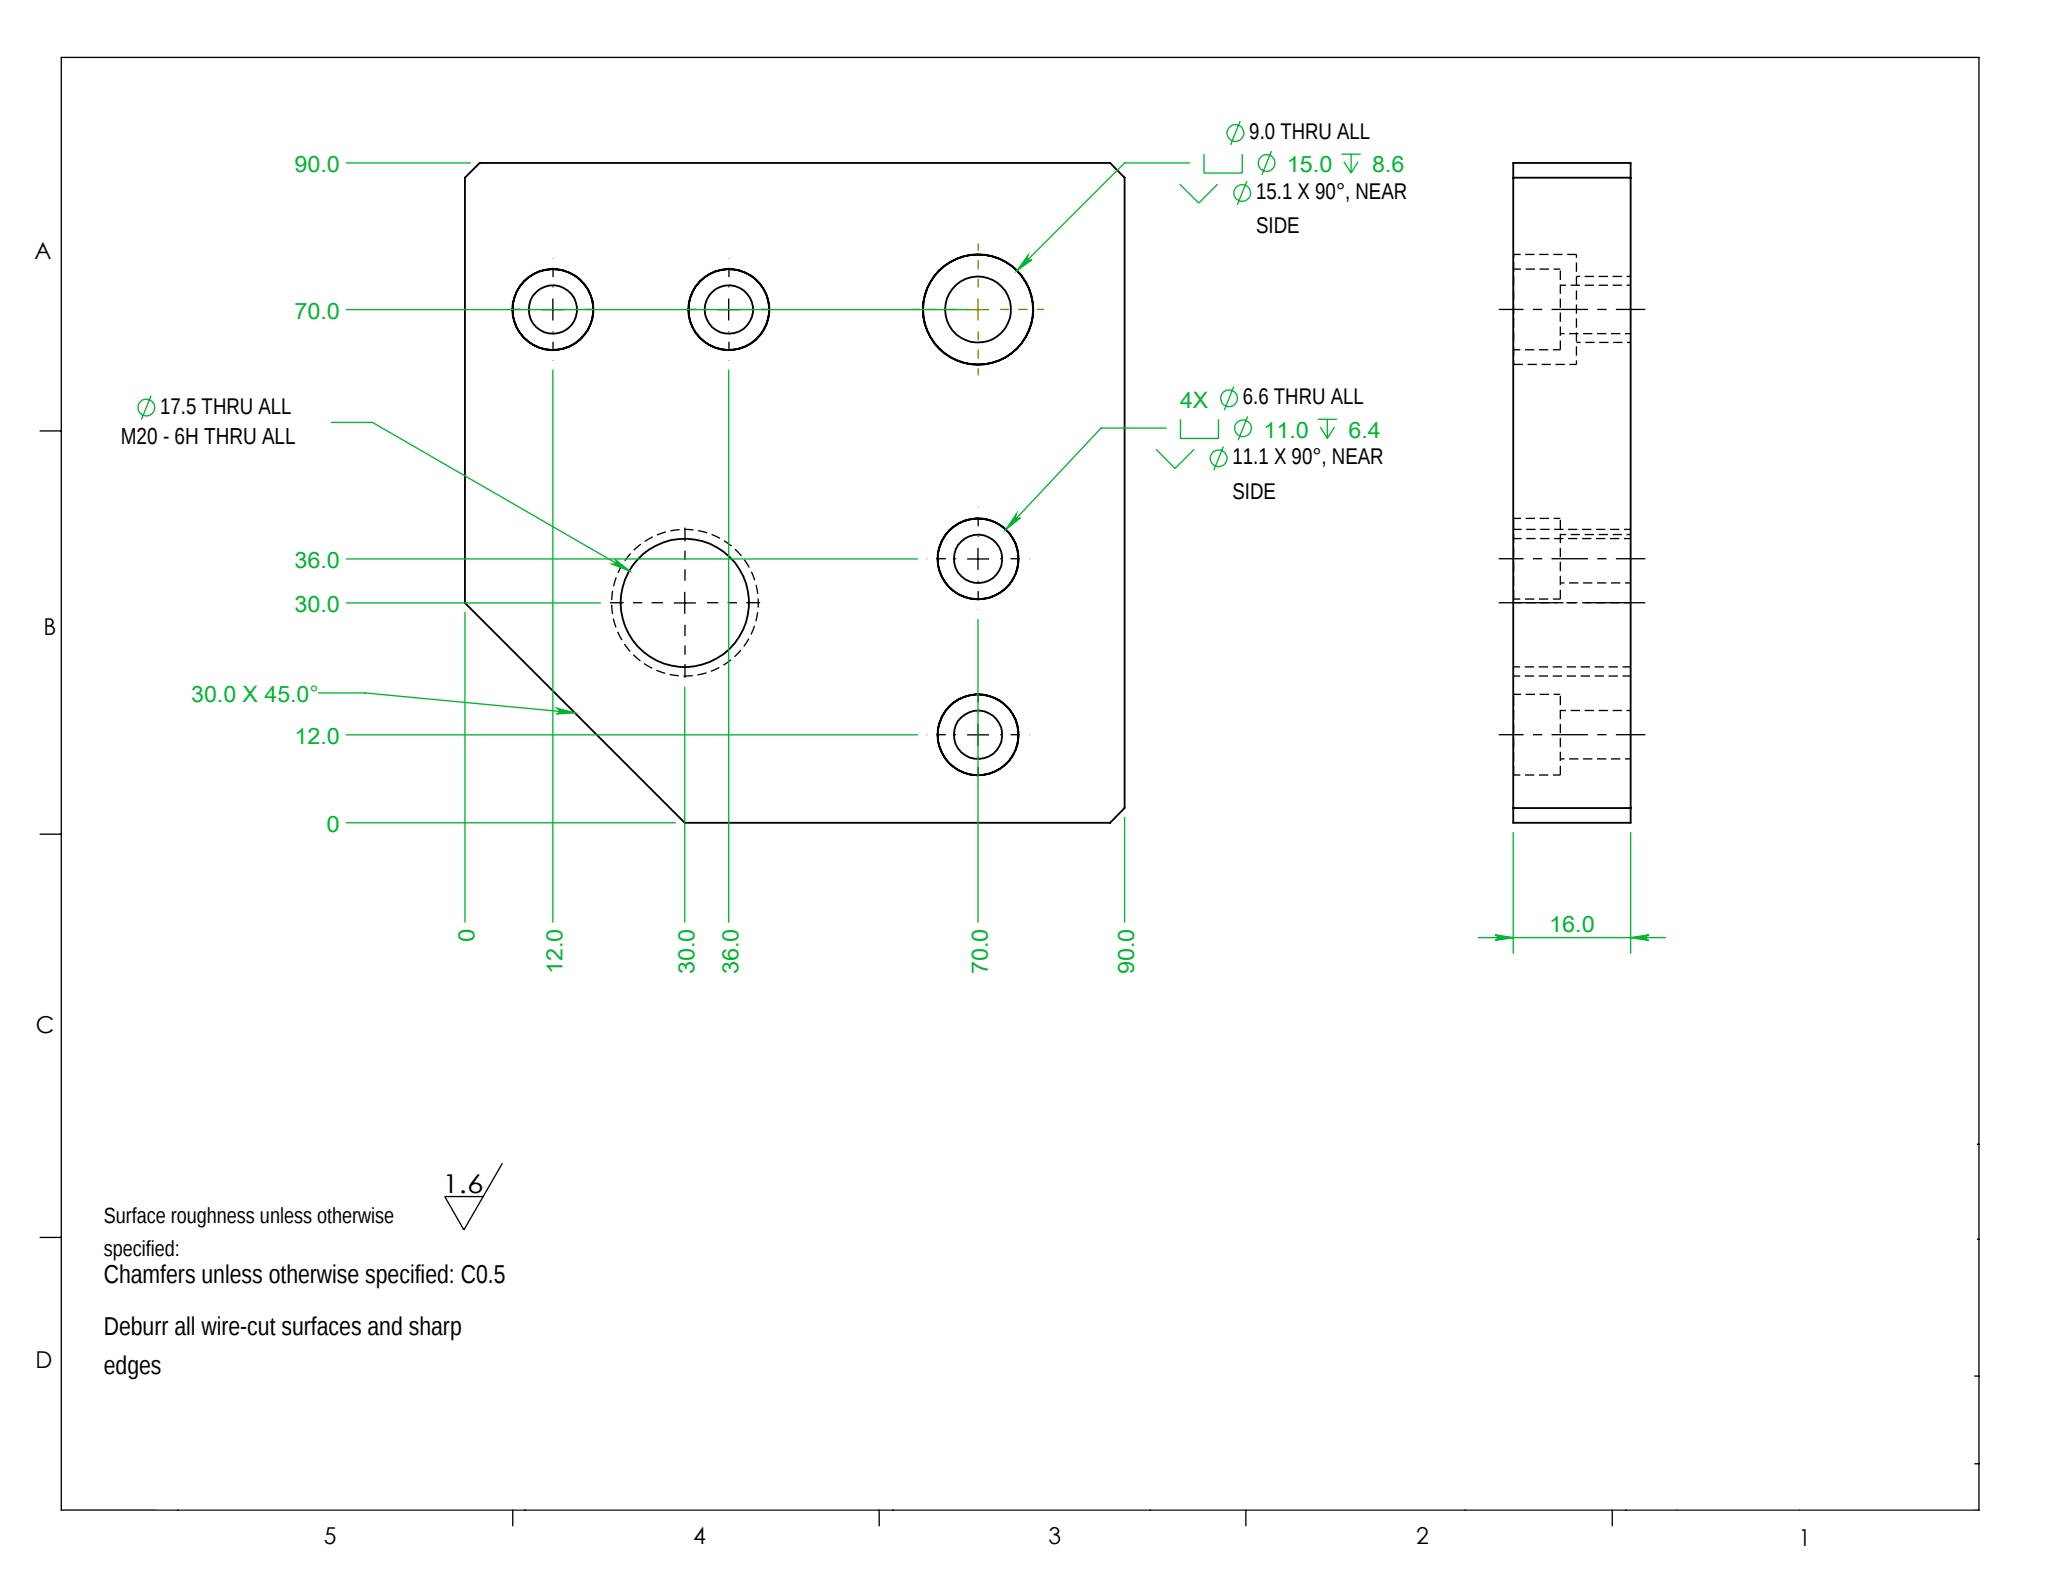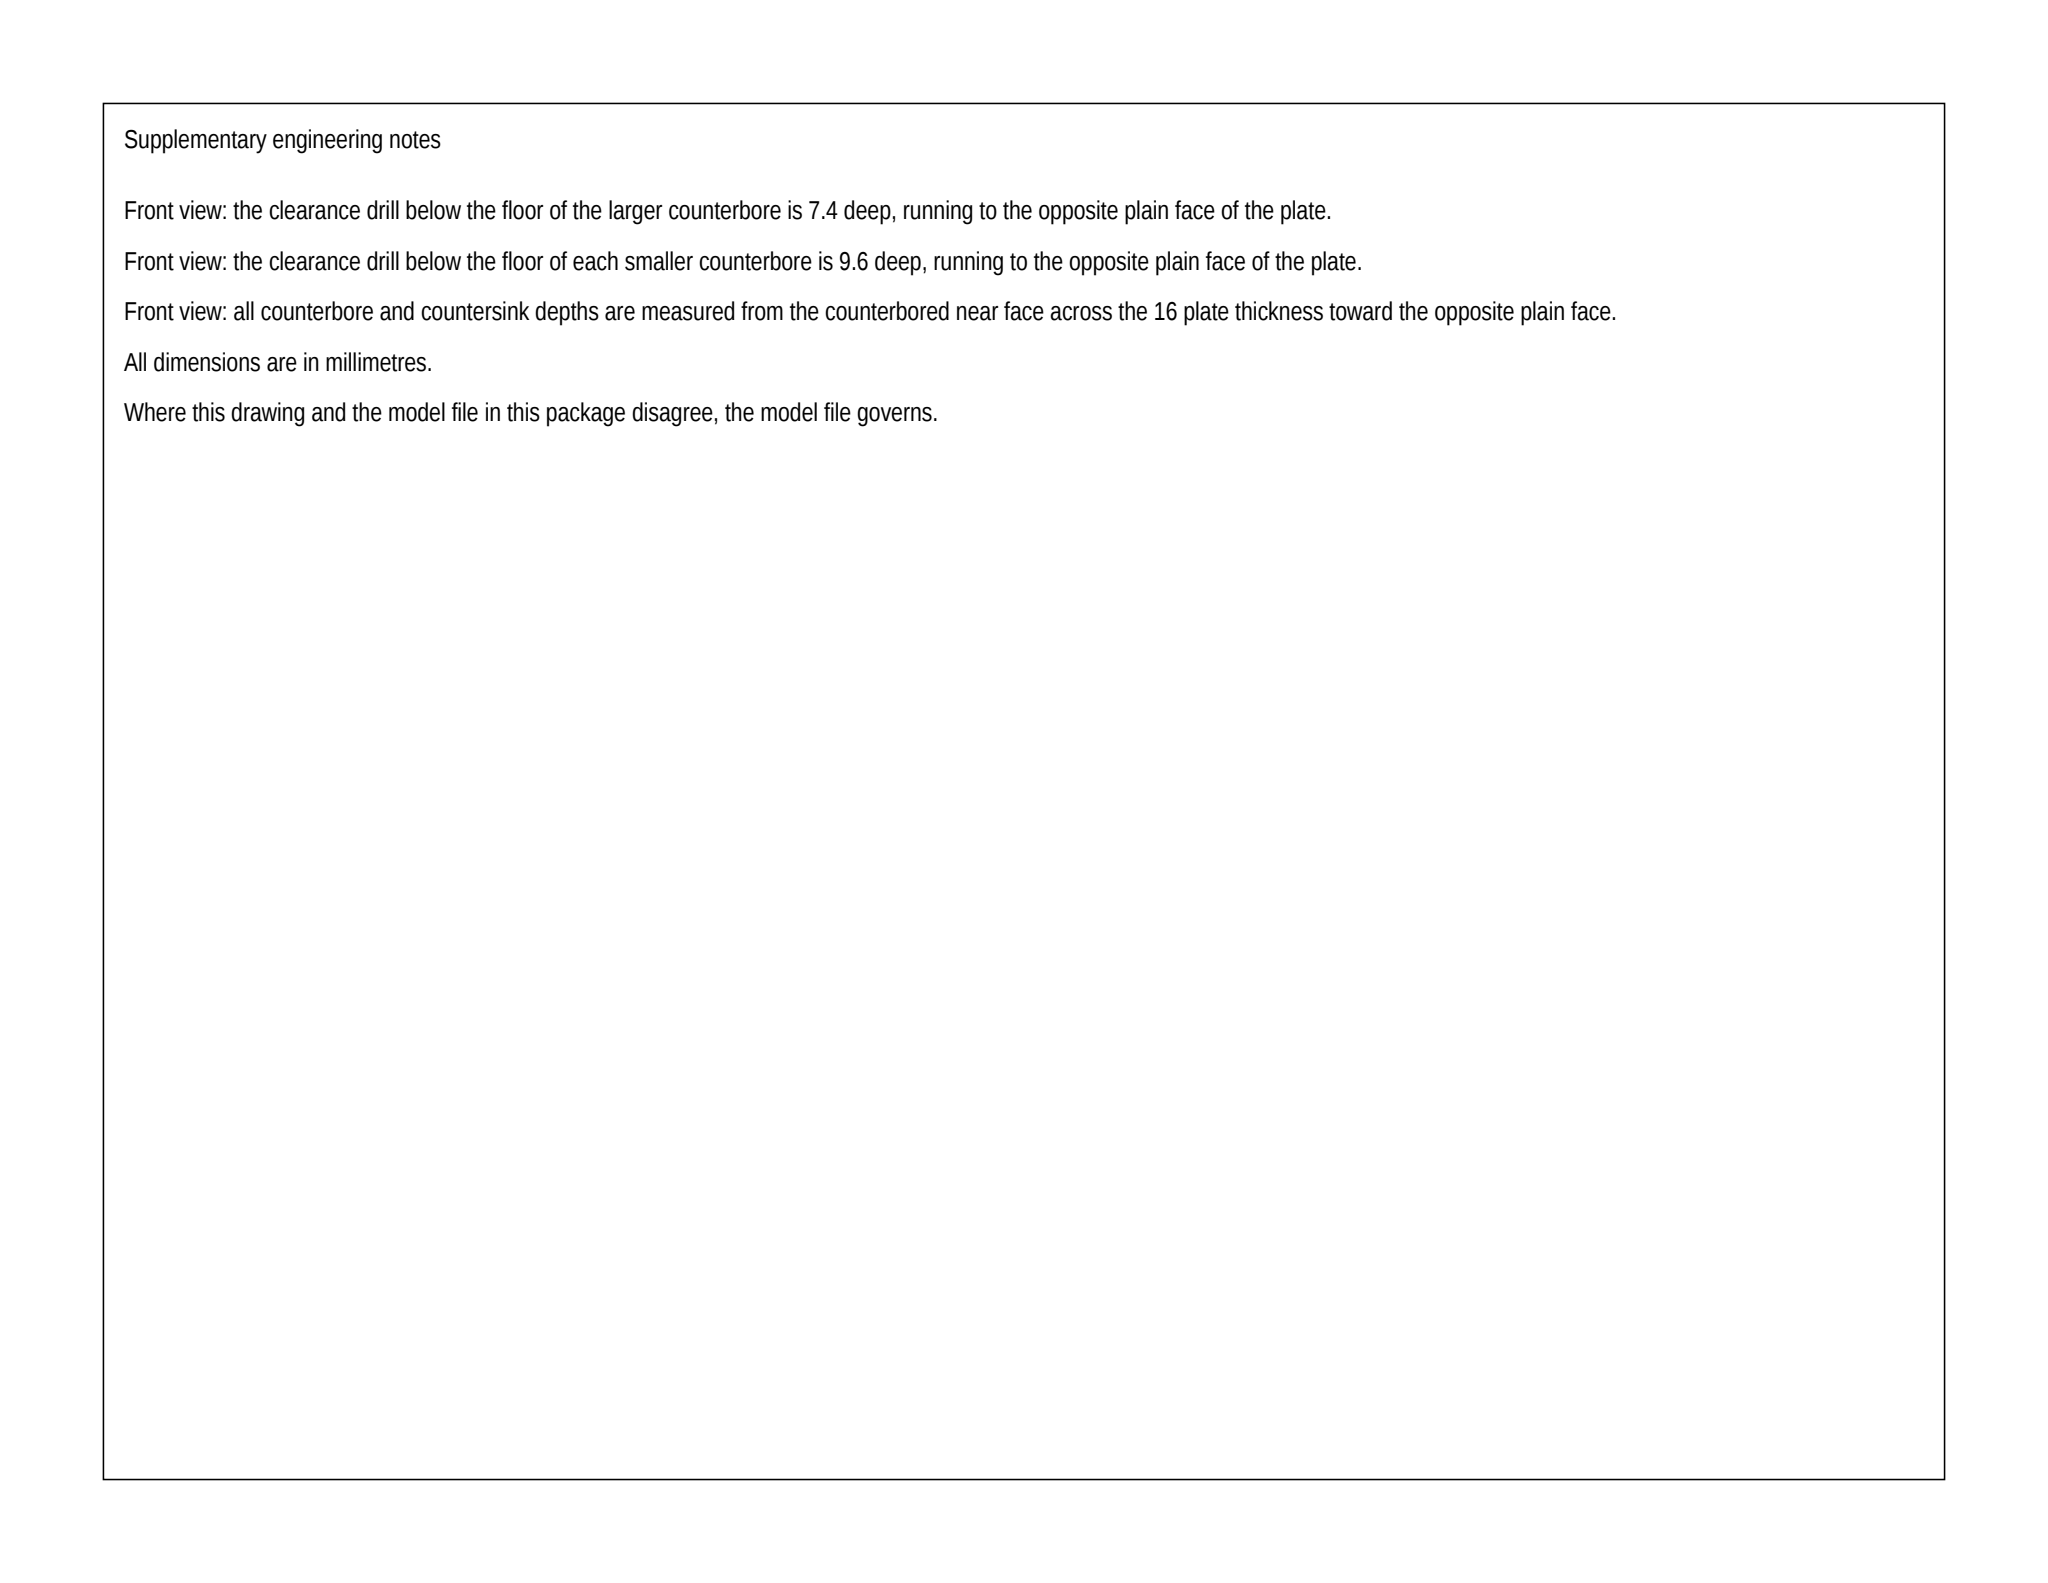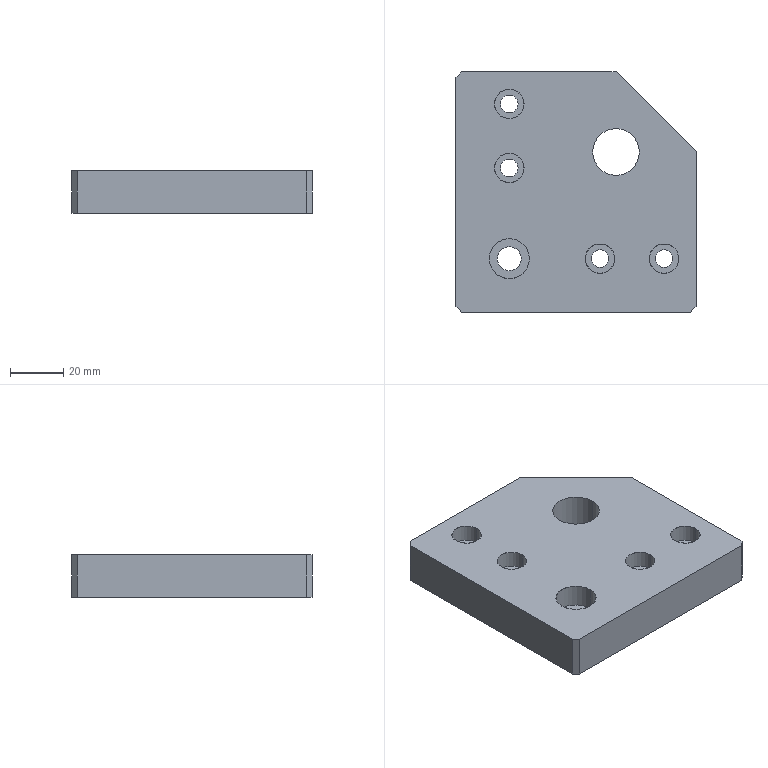Part | SolidWorks | mm | 1 solid | 47 faces | box 90 x 90 x 16 mm | volume 112718 mm3 | cylinder 22 | plane 15 | cone 10 | commonest cylinder face diameters 11 x8 6.6 x8 15 x2 9 x2 17.5 x2
build123d program:
from build123d import *

# Parameters (mm, degrees)
SKETCH1_W                                      = 90
SKETCH1_H                                      = 90
BOSS_EXTRUDE1_DEPTH                            = 16
M6_HEX_SOCKET_HEAD_CAP_SCREW_CBORE1_AT_2_COUNT = 2
M6_HEX_SOCKET_HEAD_CAP_SCREW_CBORE1_AT_2_PITCH = 48.083
M6_HEX_SOCKET_HEAD_CAP_SCREW_CBORE1_AT_3_COUNT = 2
M6_HEX_SOCKET_HEAD_CAP_SCREW_CBORE1_AT_3_PITCH = 67.231
M6_HEX_SOCKET_HEAD_CAP_SCREW_CBORE1_AT_4_COUNT = 2
M6_HEX_SOCKET_HEAD_CAP_SCREW_CBORE1_AT_4_PITCH = 24
CHAMFER1_SIZE                                  = 2
M20_TAPPED_HOLE1_D                             = 17.5
CHAMFER3_SIZE                                  = 30


with BuildPart() as part:
    # Sketch1 → Boss-Extrude1 (new body)
    with BuildSketch(Plane.XY):
        with Locations((45, 45)):
            Rectangle(SKETCH1_W, SKETCH1_H)
    extrude(amount=BOSS_EXTRUDE1_DEPTH)

    # Sketch3 → M6 Hex Socket Head Cap Screw CBORE1 (revolve, cut)
    with BuildSketch(Plane(origin=(20, 54, 16), x_dir=(0, -1, 0), z_dir=(1, 0, 0))):
        Polygon((0, 0), (0, 16), (3.3, 16), (3.3, 6.4), (5.5, 6.4), (5.5, 0.025), (5.525, 0), align=None)
    m6_hex_socket_head_cap_screw_cbore1 = revolve(axis=Axis((20, 54, 22.35), (0, 0, -1)), mode=Mode.SUBTRACT)

    # M6 Hex Socket Head Cap Screw CBORE1 at 2: M6 Hex Socket Head Cap Screw CBORE1 ×2
    with Locations(*[Vector(0.7071, -0.7071, 0) * (i * M6_HEX_SOCKET_HEAD_CAP_SCREW_CBORE1_AT_2_PITCH) for i in range(1, M6_HEX_SOCKET_HEAD_CAP_SCREW_CBORE1_AT_2_COUNT)]):
        add(m6_hex_socket_head_cap_screw_cbore1, mode=Mode.SUBTRACT)

    # M6 Hex Socket Head Cap Screw CBORE1 at 3: M6 Hex Socket Head Cap Screw CBORE1 ×2
    with Locations(*[Vector(0.8627, -0.5057, 0) * (i * M6_HEX_SOCKET_HEAD_CAP_SCREW_CBORE1_AT_3_PITCH) for i in range(1, M6_HEX_SOCKET_HEAD_CAP_SCREW_CBORE1_AT_3_COUNT)]):
        add(m6_hex_socket_head_cap_screw_cbore1, mode=Mode.SUBTRACT)

    # M6 Hex Socket Head Cap Screw CBORE1 at 4: M6 Hex Socket Head Cap Screw CBORE1 ×2
    with Locations(*[(0, i * M6_HEX_SOCKET_HEAD_CAP_SCREW_CBORE1_AT_4_PITCH, 0) for i in range(1, M6_HEX_SOCKET_HEAD_CAP_SCREW_CBORE1_AT_4_COUNT)]):
        add(m6_hex_socket_head_cap_screw_cbore1, mode=Mode.SUBTRACT)

    # Chamfer1
    chamfer1_edges = [part.edges().sort_by_distance(p)[0] for p in [
        (0, 90, 8),
        (90, 0, 8),
        (0, 0, 8),
    ]]
    chamfer(chamfer1_edges, length=CHAMFER1_SIZE)

    # M20 Tapped Hole1 (through all)
    with Locations(Plane.XY.offset(16)):
        with Locations((60, 60)):
            Hole(M20_TAPPED_HOLE1_D / 2)

    # Chamfer3
    chamfer3_edges = [part.edges().sort_by_distance(p)[0] for p in [
        (90, 90, 8),
    ]]
    chamfer(chamfer3_edges, length=CHAMFER3_SIZE)

    # Sketch8 → M8 Hex Socket Head Cap Screw CBORE2 (revolve, cut)
    with BuildSketch(Plane(origin=(20, 20, 16), x_dir=(0, -1, 0), z_dir=(1, 0, 0))):
        Polygon((0, 0), (0, 16), (4.5, 16), (4.5, 8.6), (7.5, 8.6), (7.5, 0.025), (7.525, 0), align=None)
    revolve(axis=Axis((20, 20, 22.35), (0, 0, -1)), mode=Mode.SUBTRACT)


solid = part.part